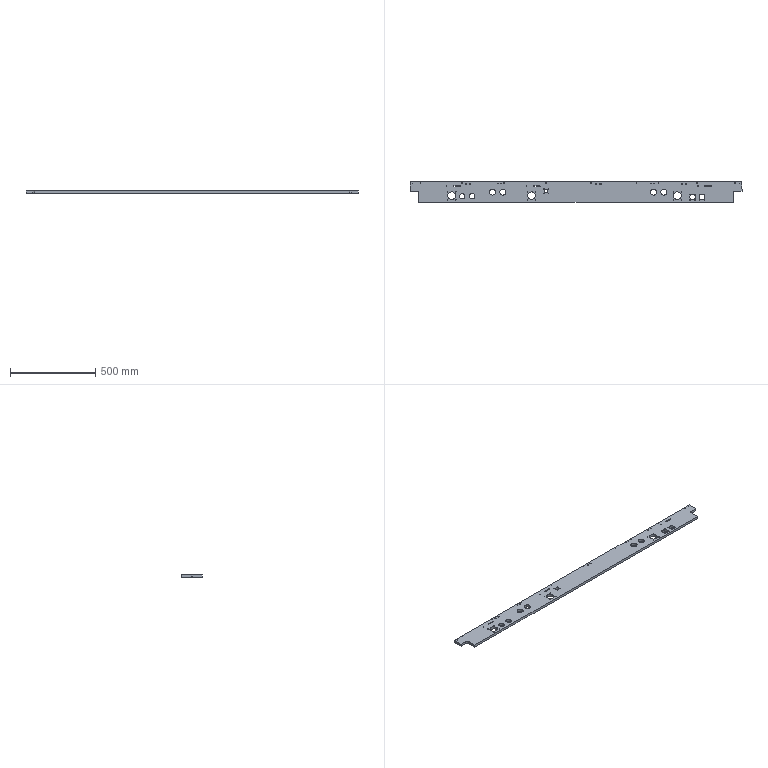Component | SolidWorks | SL010-LeftStreamline-1-1_SL010-LXFB-010203-002-1-1 | 1 solid | 231 faces | volume 3176691 mm3 | cylinder 176 | plane 31 | cone 24 | commonest cylinder face diameters 3.3 x42 4.2 x42 2.5 x24 8 x12 4.5 x12 10 x9 5.5 x9 32 x8 | material Aluminum-6061